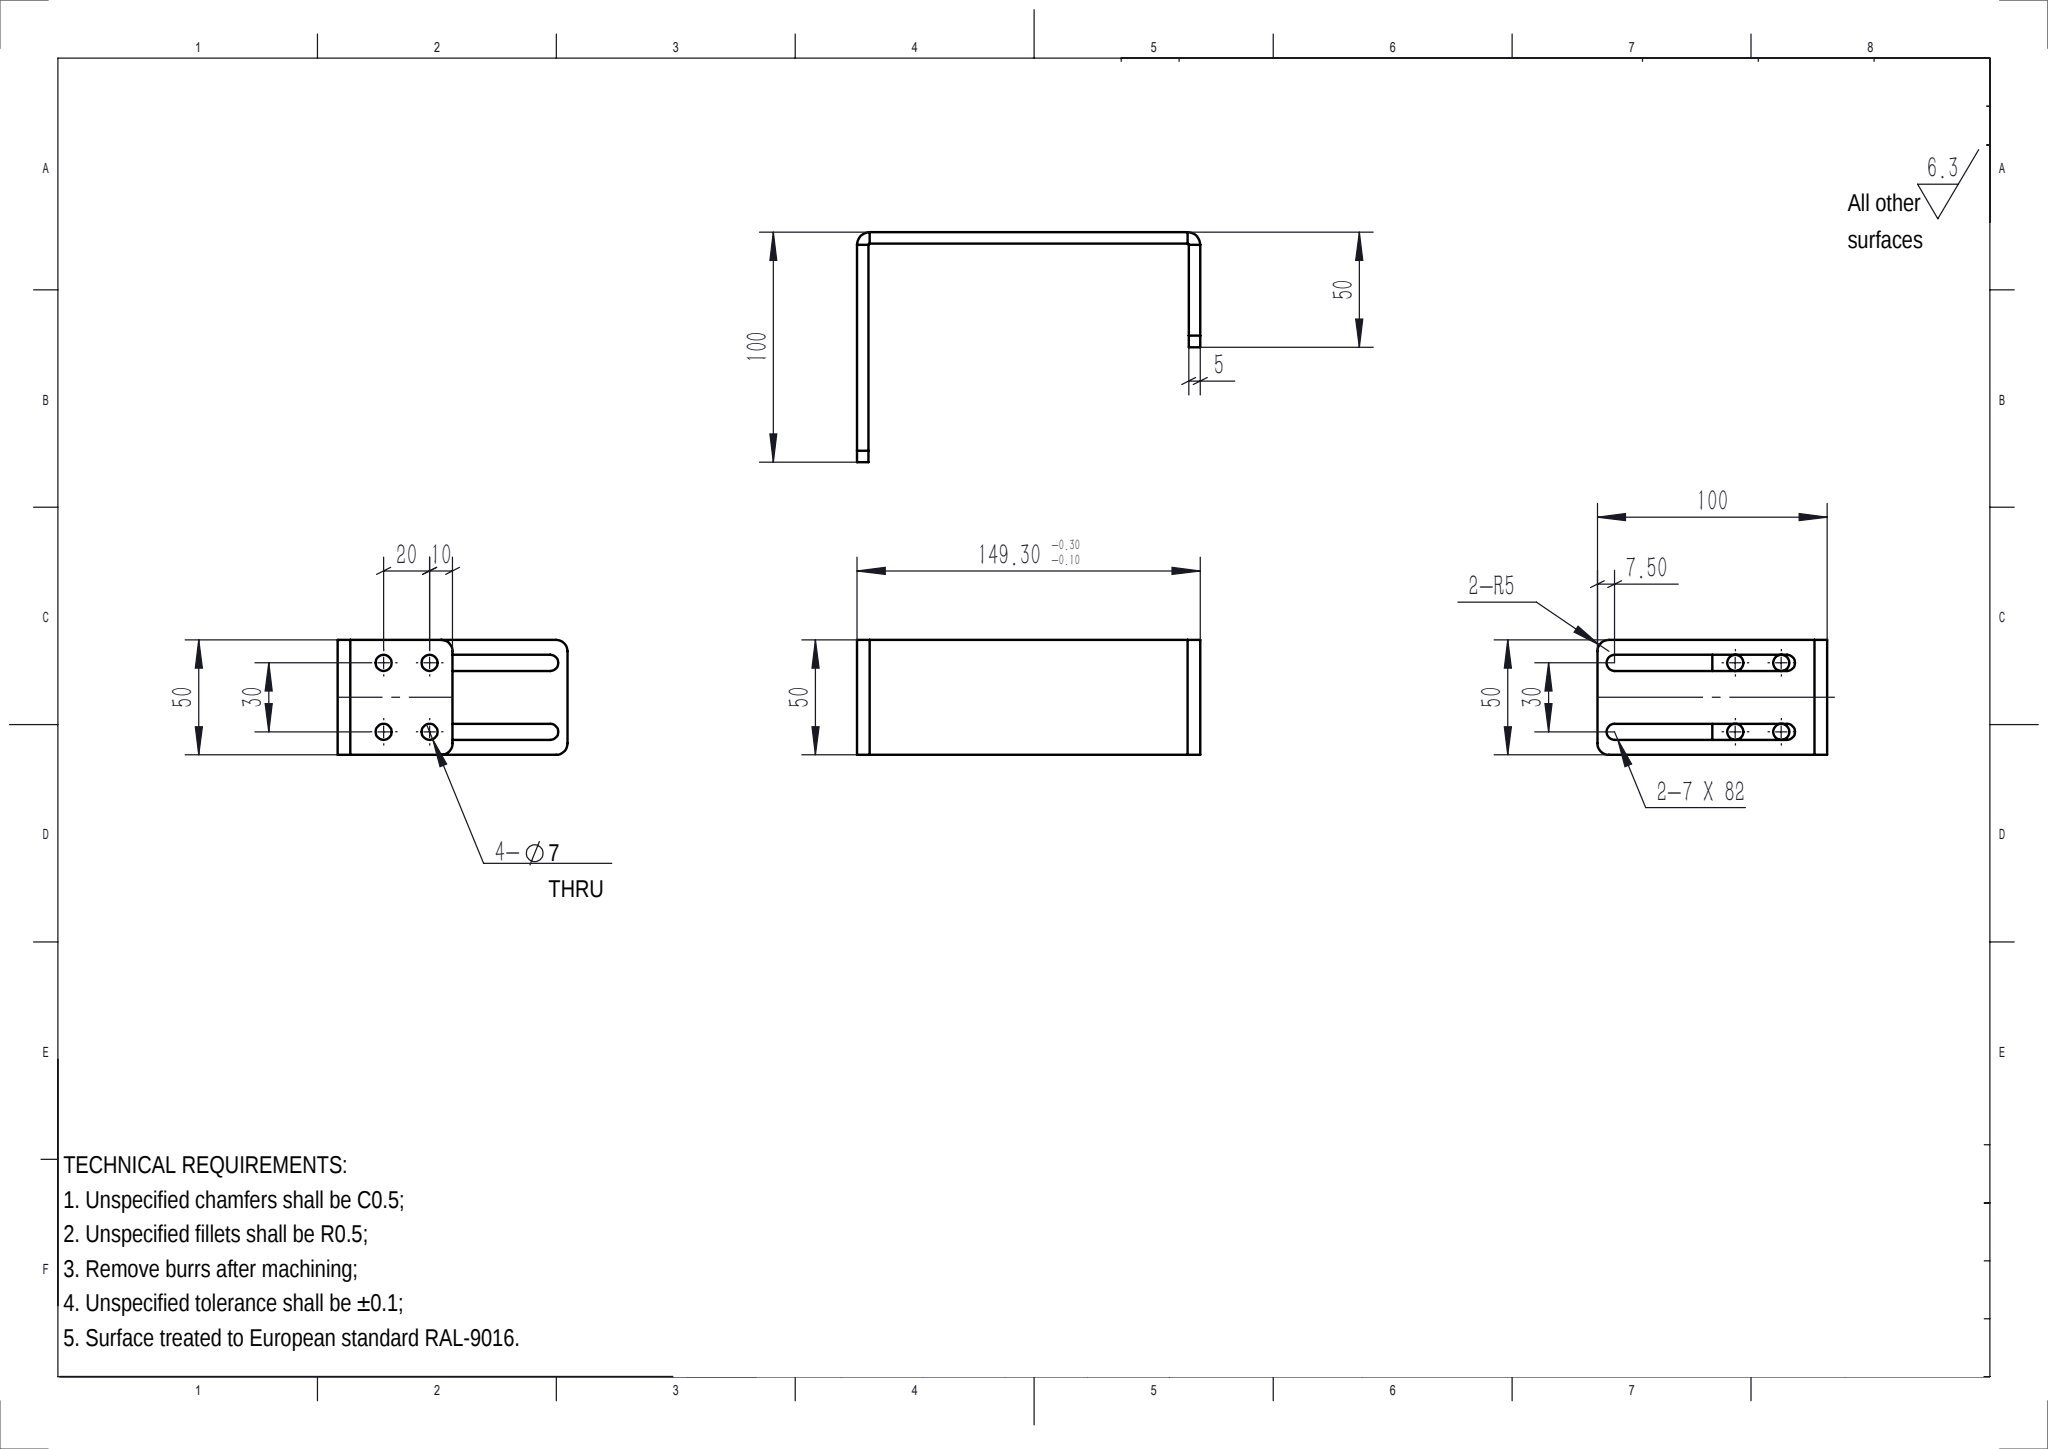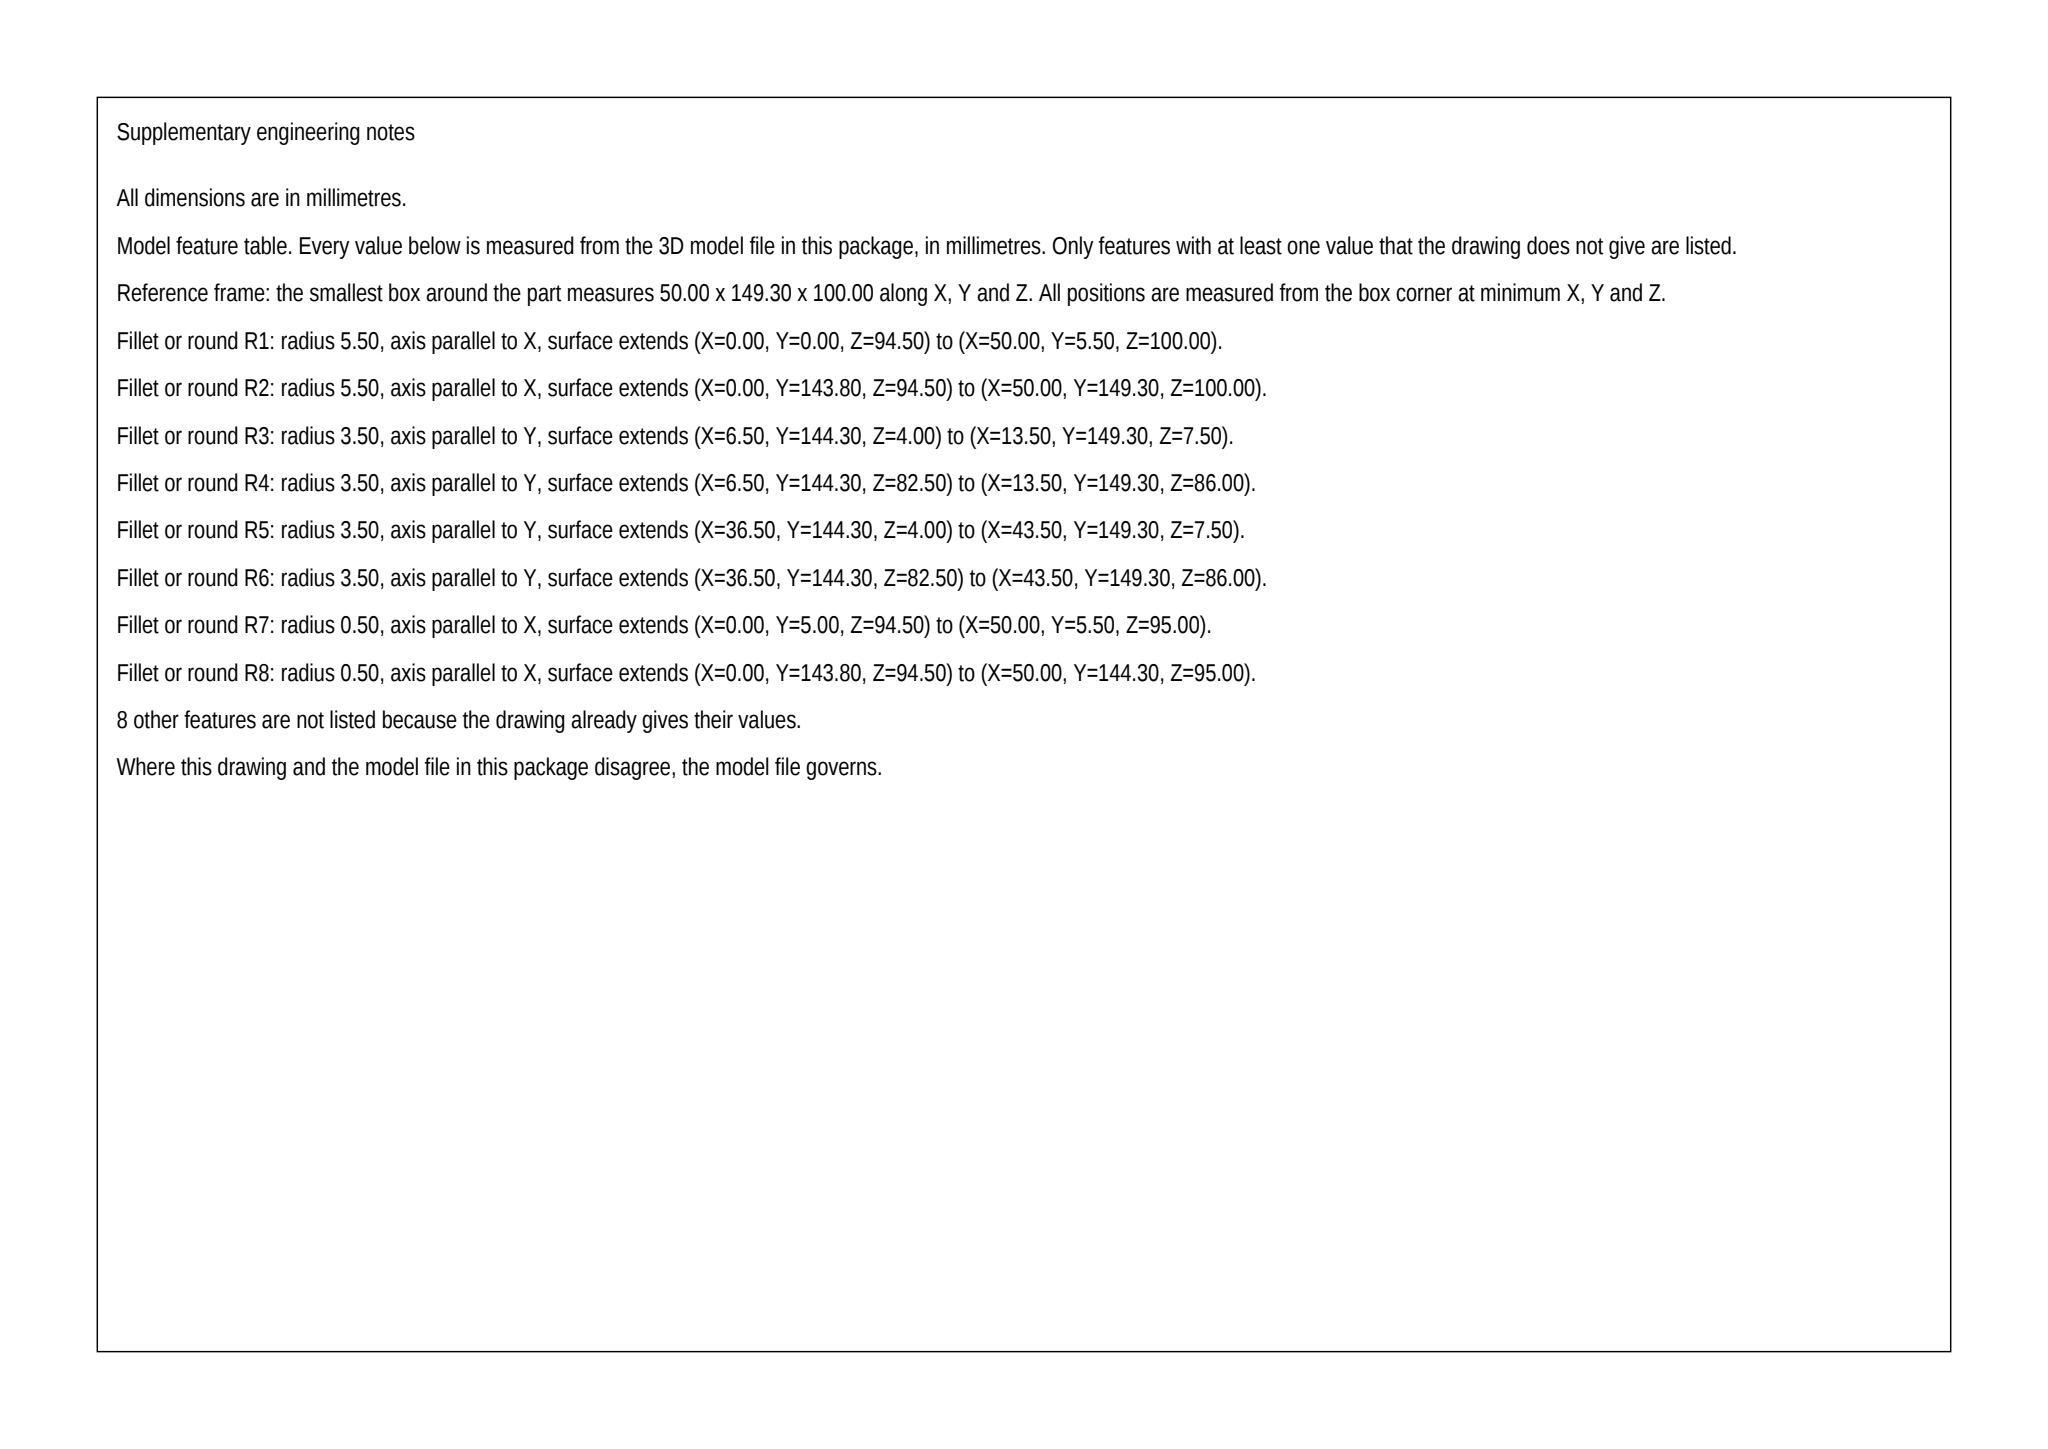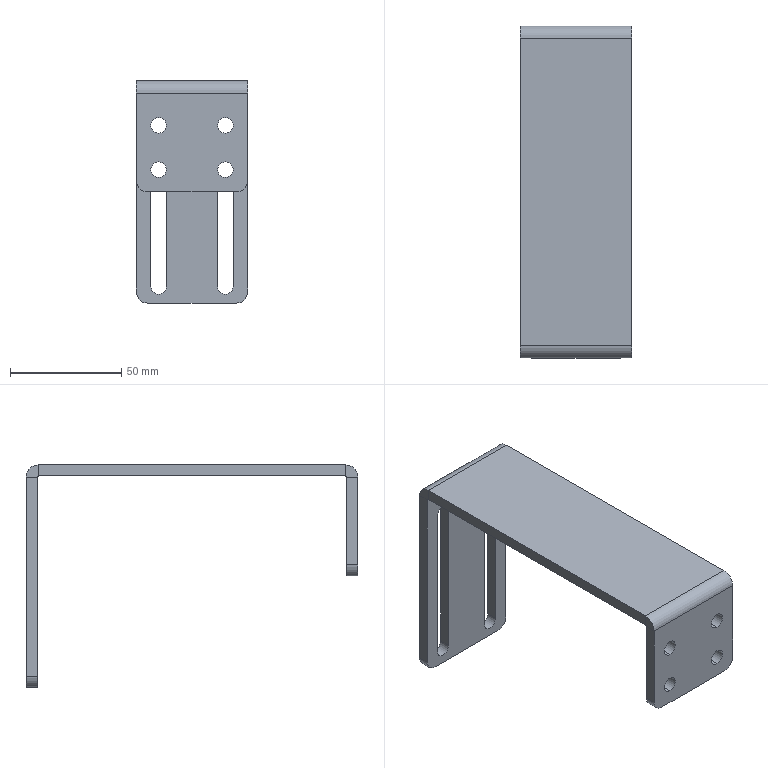Part | SolidWorks | mm | 1 solid | 44 faces | box 50 x 149.3 x 100 mm | volume 65169 mm3 | cylinder 22 | plane 22 | commonest cylinder face diameters 7 x14 10 x4 11 x2 1 x2